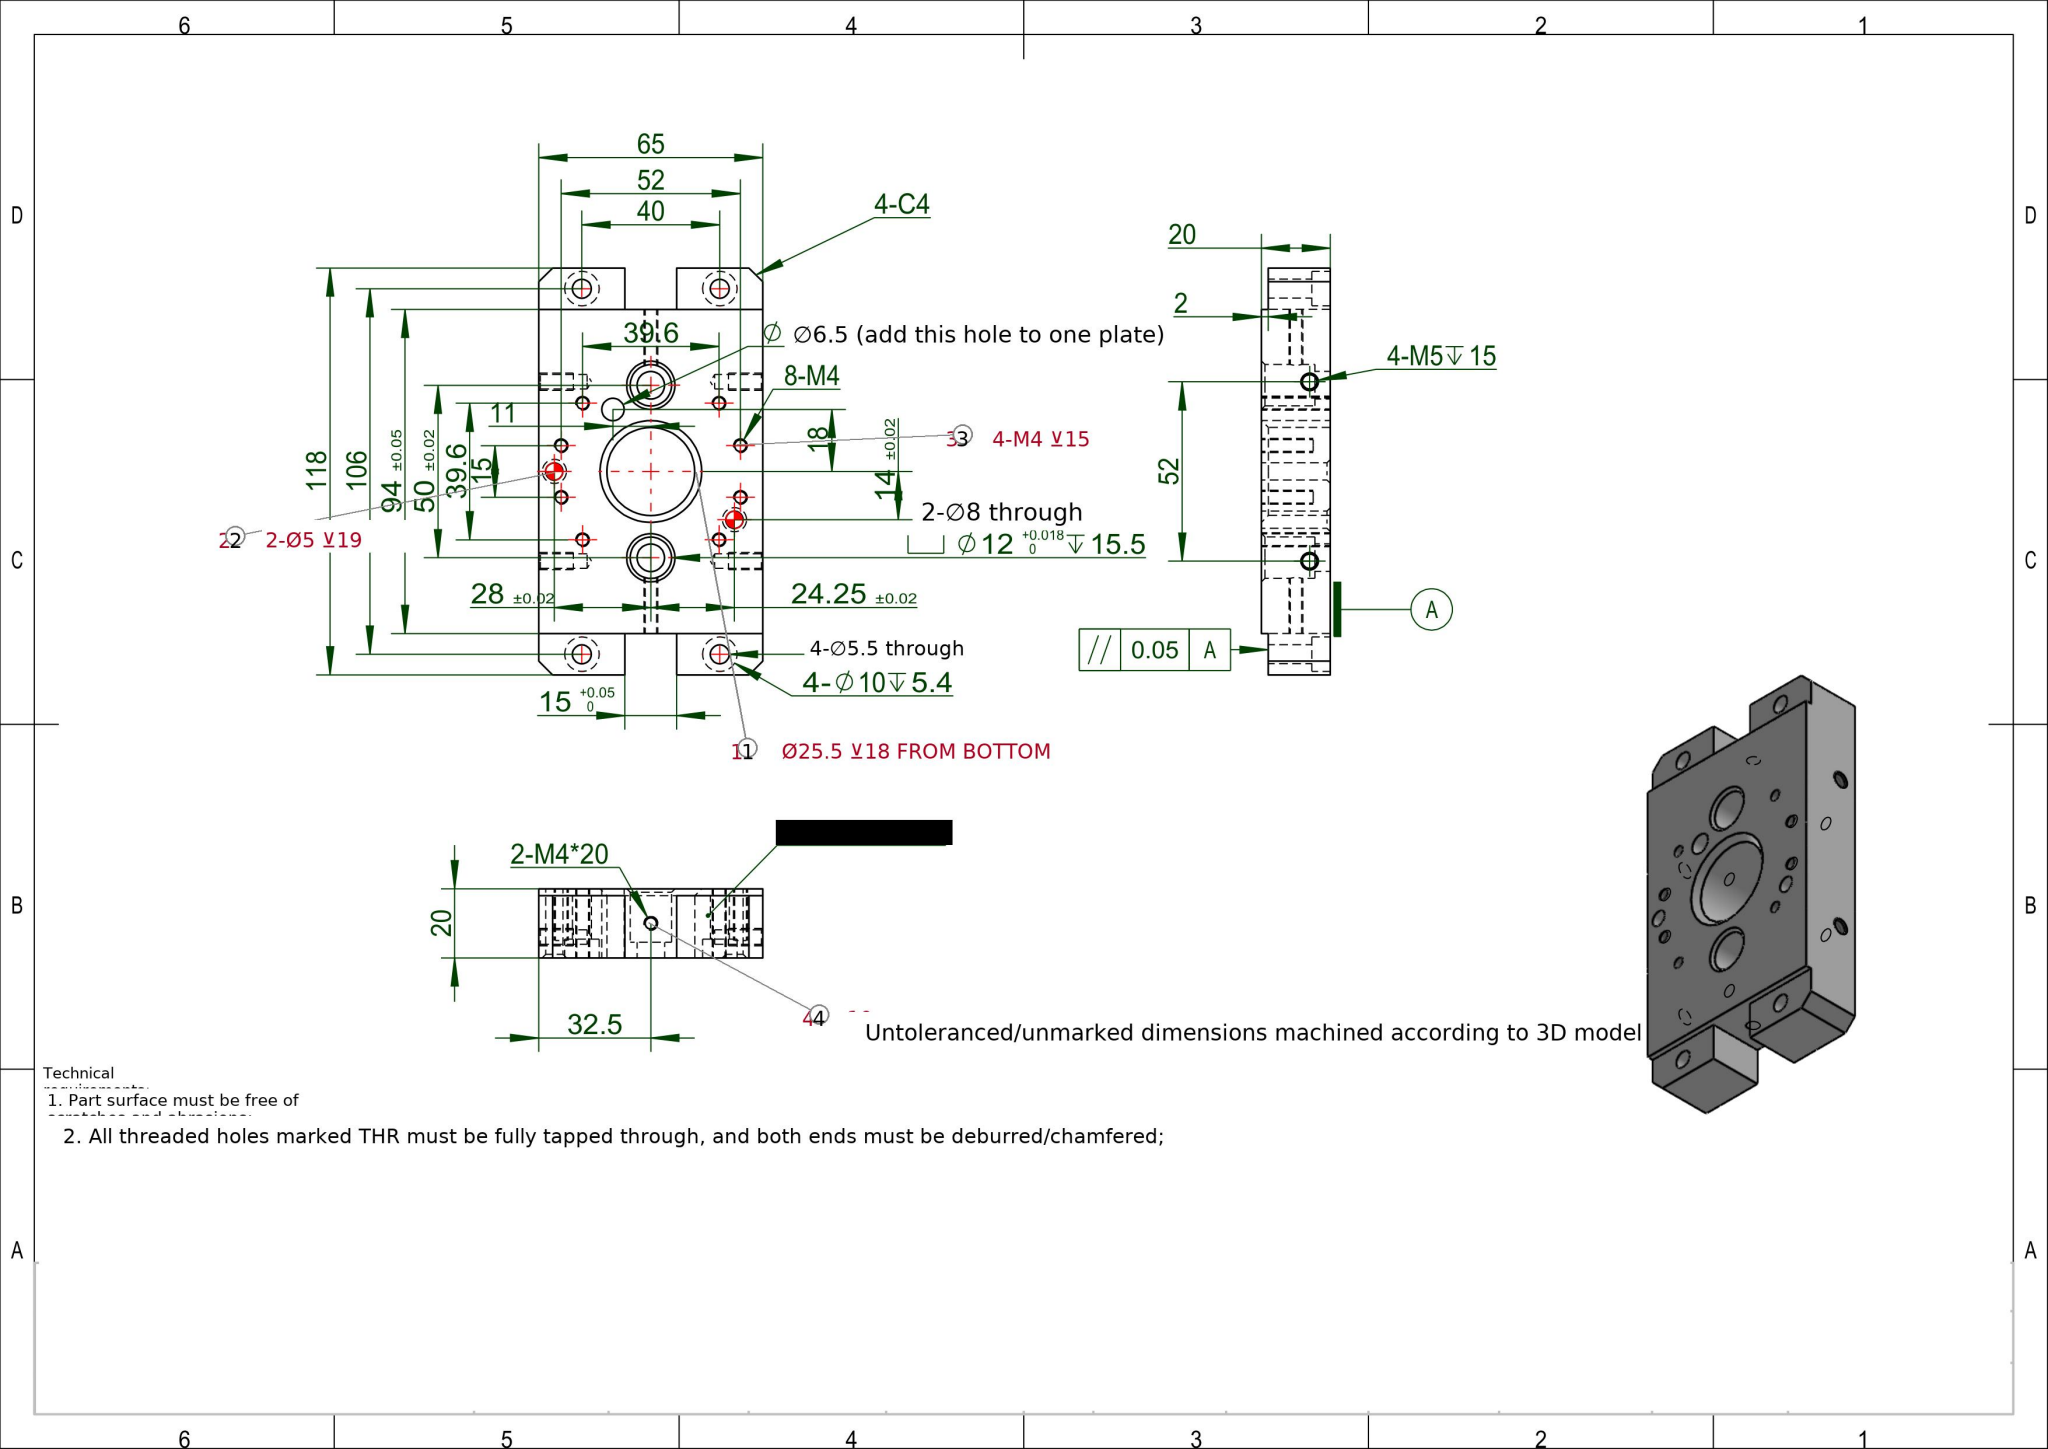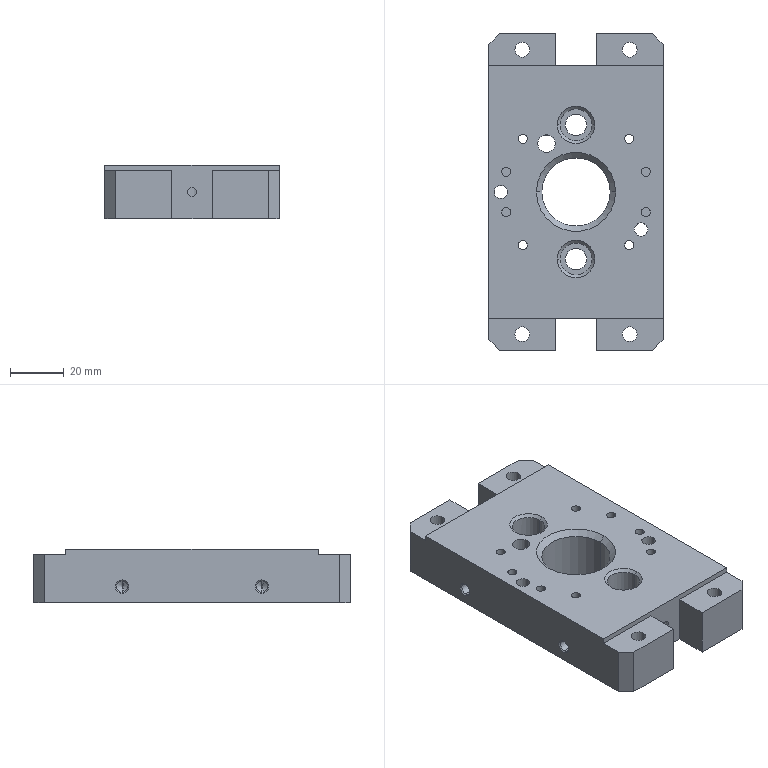Part | SolidWorks | mm | 1 solid | 118 faces | box 65 x 118 x 20 mm | volume 122132 mm3 | cylinder 60 | plane 32 | cone 26 | commonest cylinder face diameters 3.4 x16 4.2 x8 10 x8 5.5 x8 3.3 x4 12 x4 5 x4 8 x4